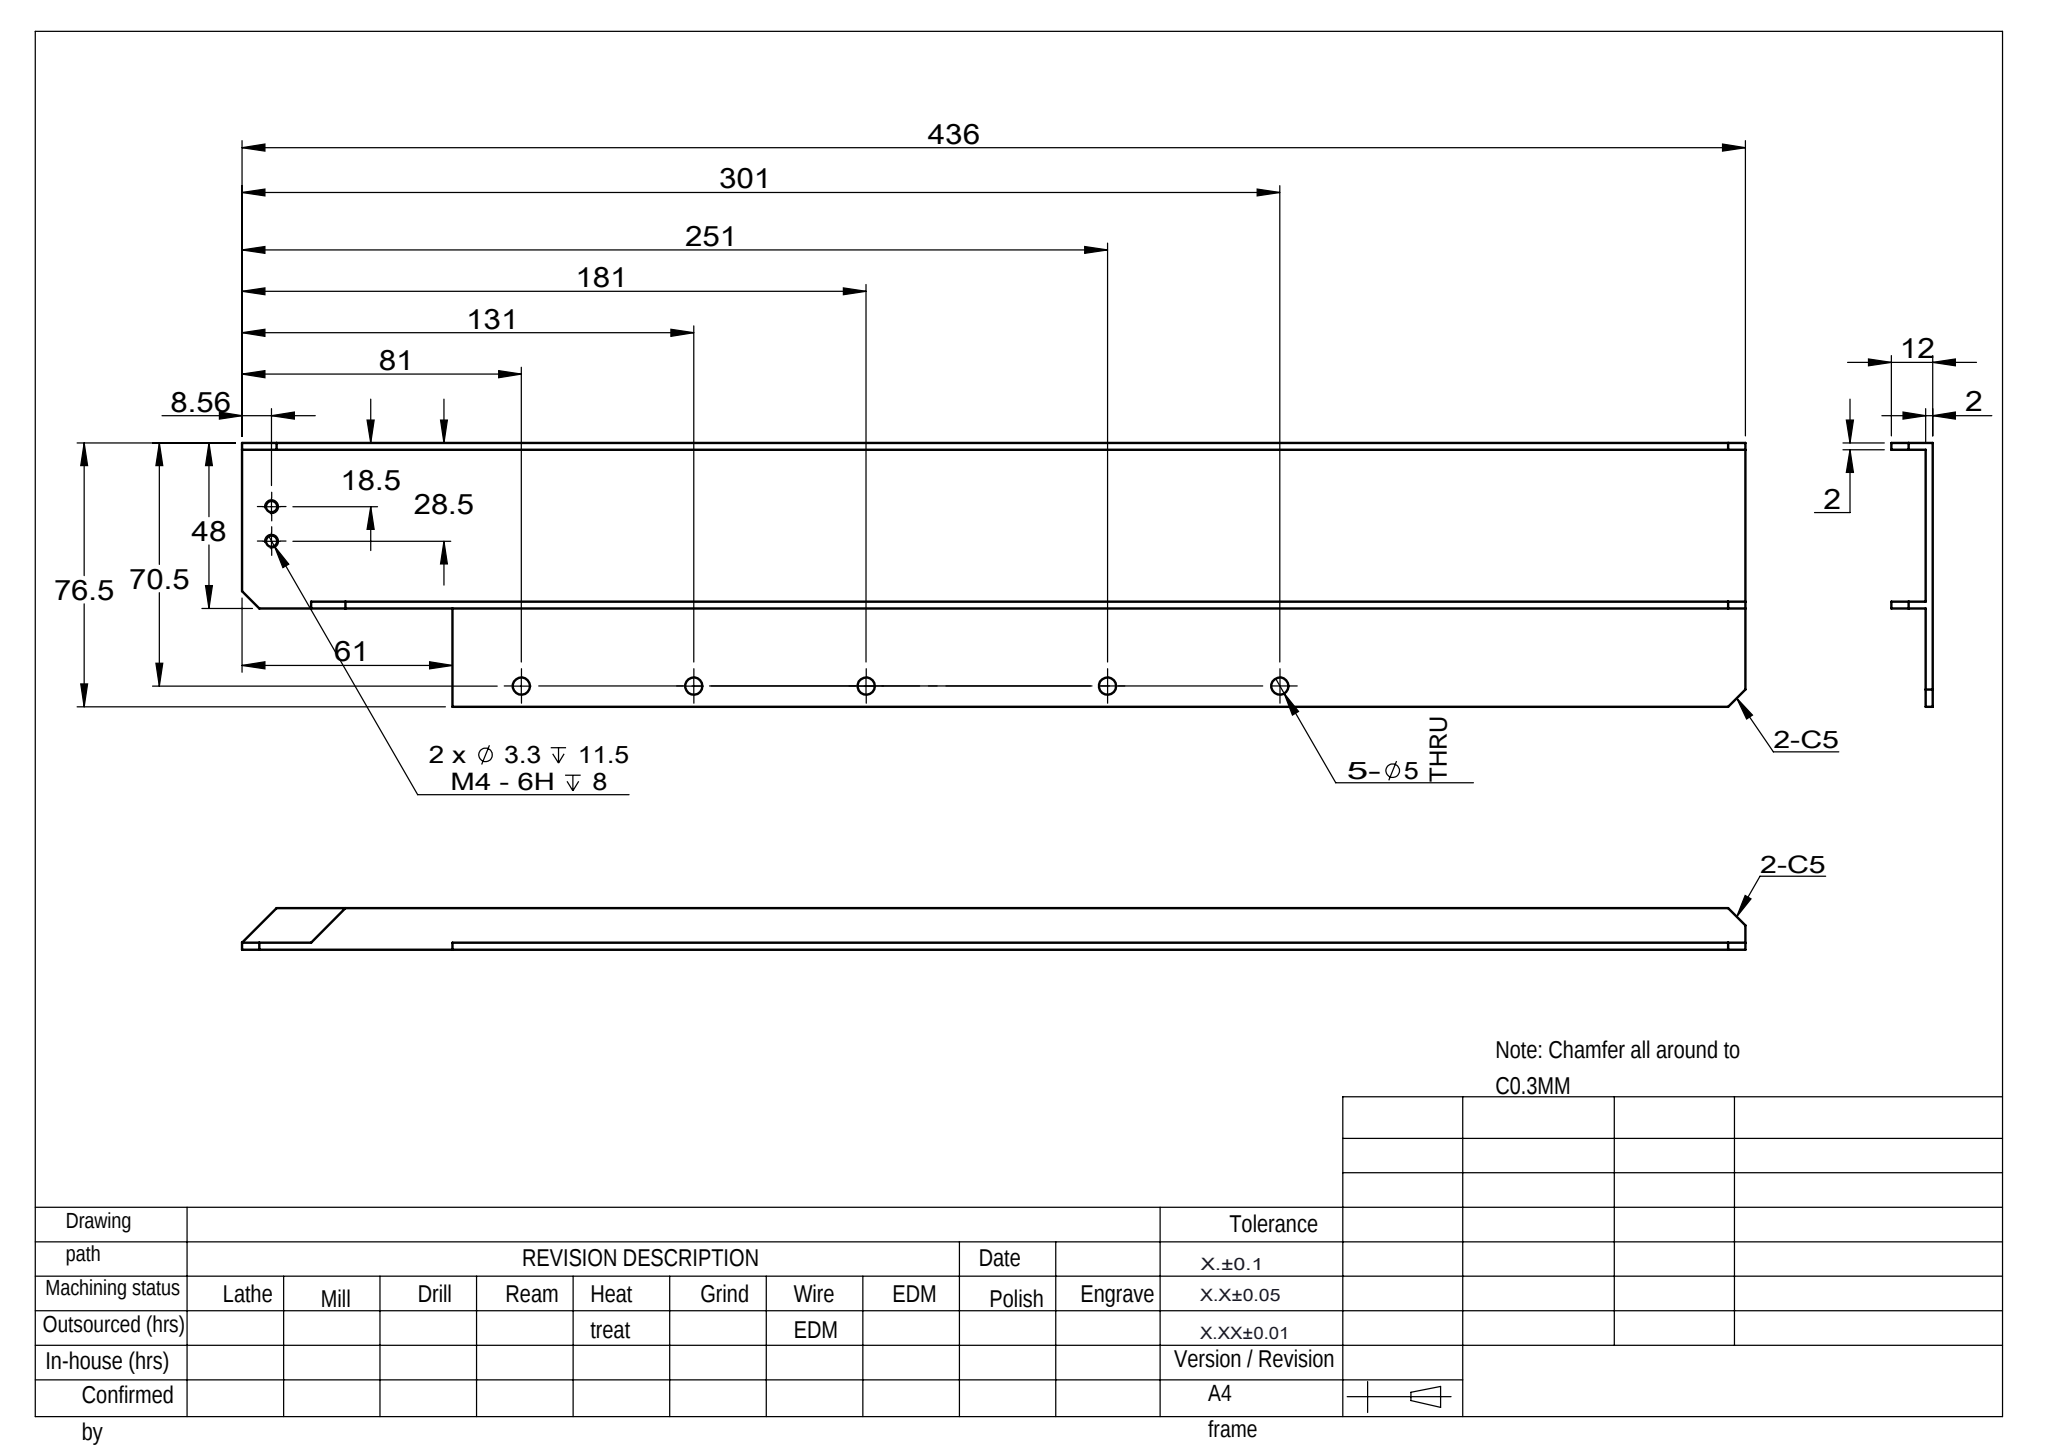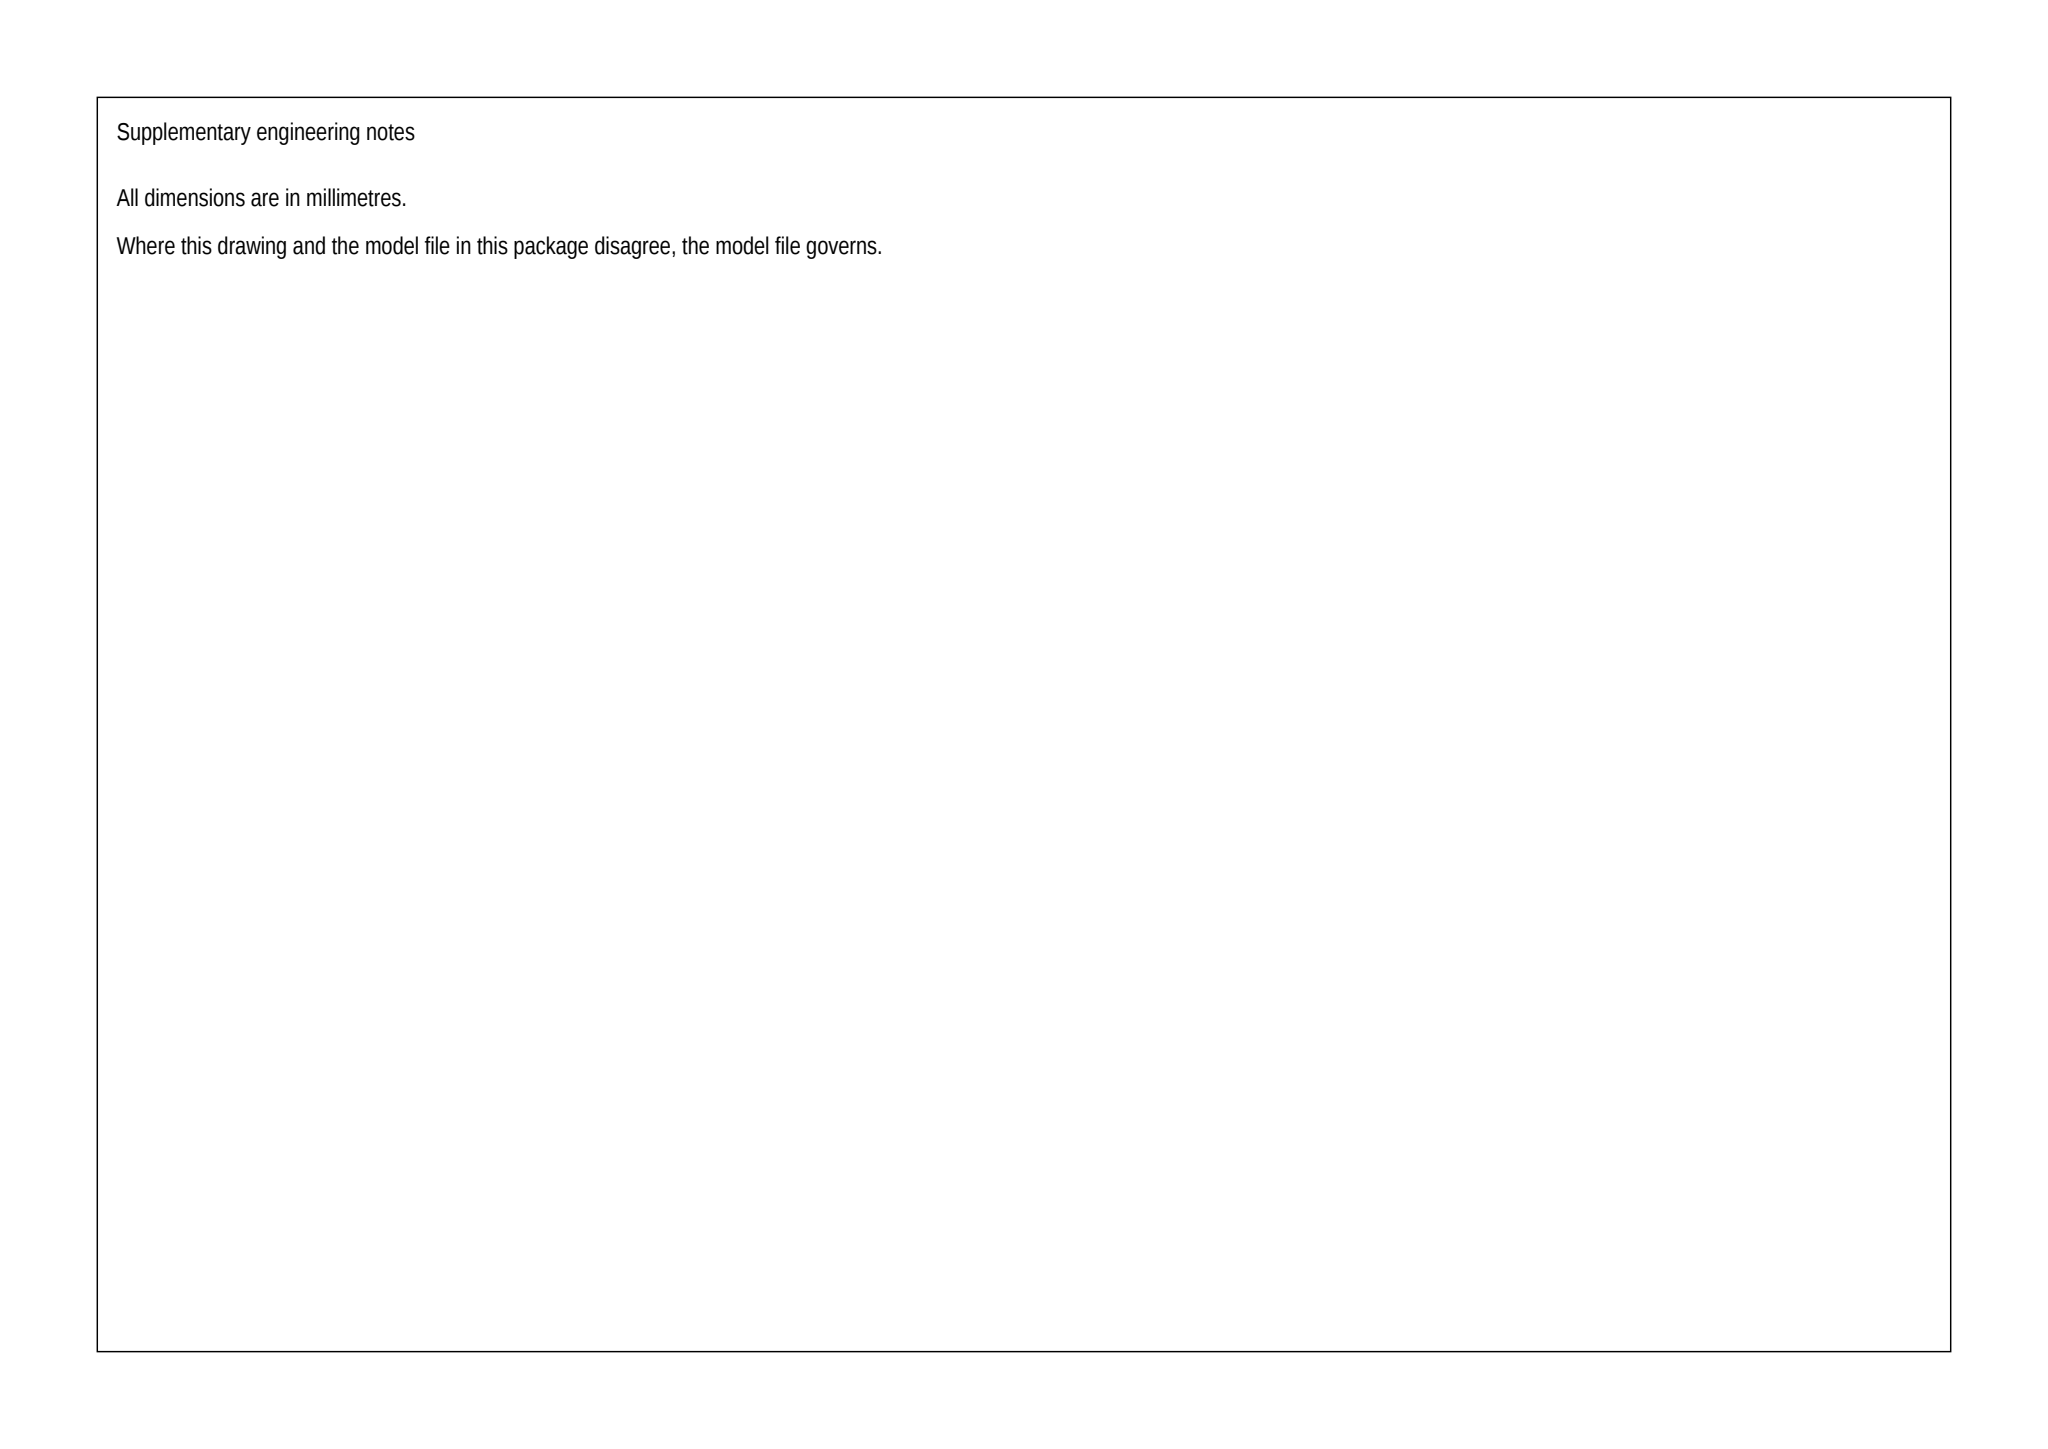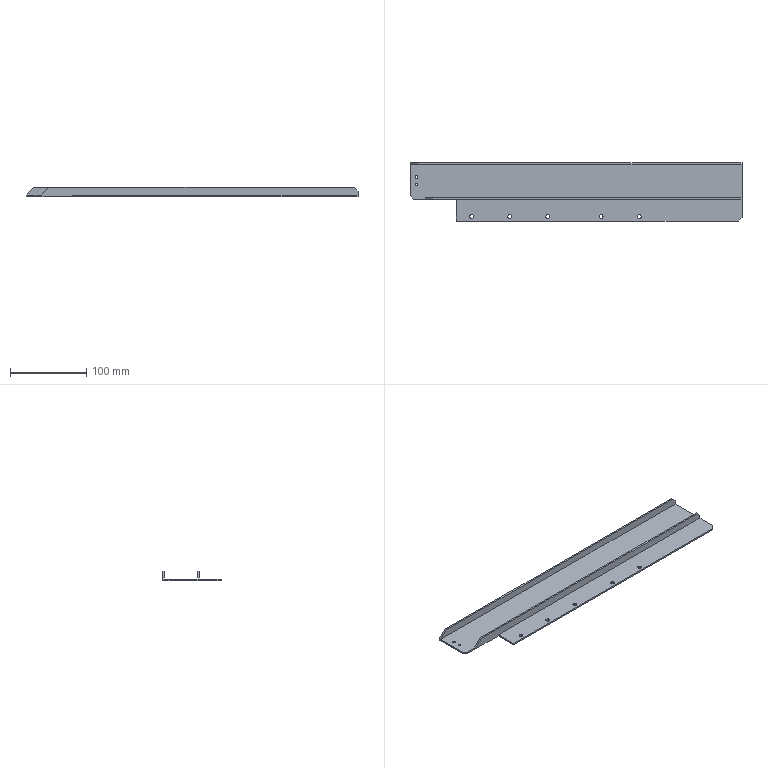Part | SolidWorks | mm | 1 solid | 33 faces | box 436 x 76.5 x 12 mm | volume 79740 mm3 | plane 19 | cylinder 14 | commonest cylinder face diameters 5 x10 3.3 x4